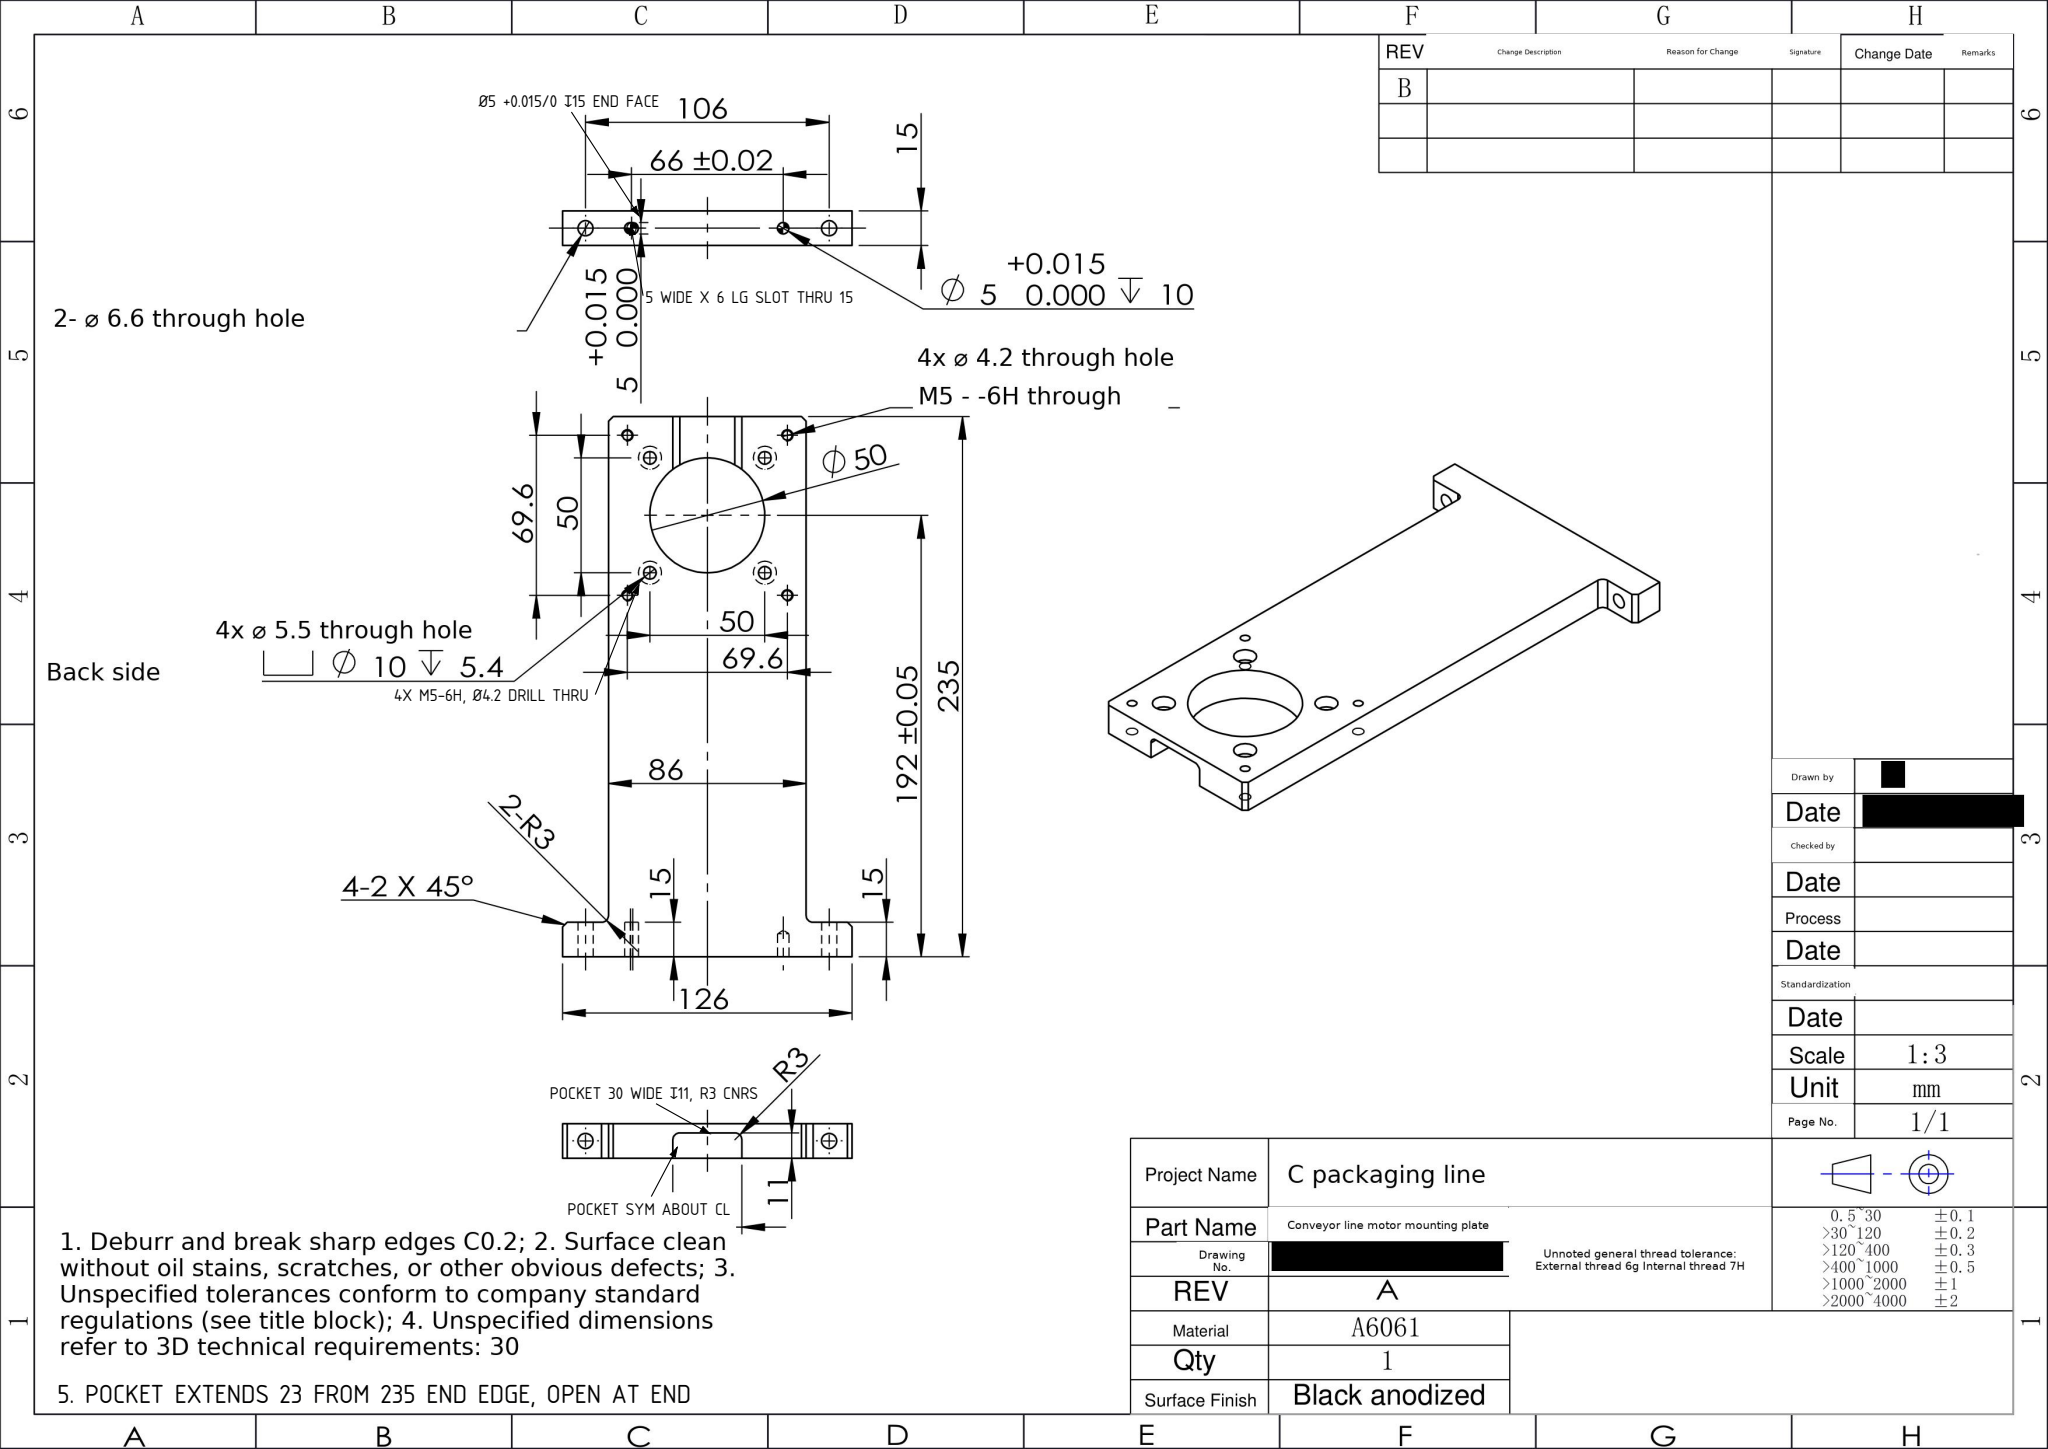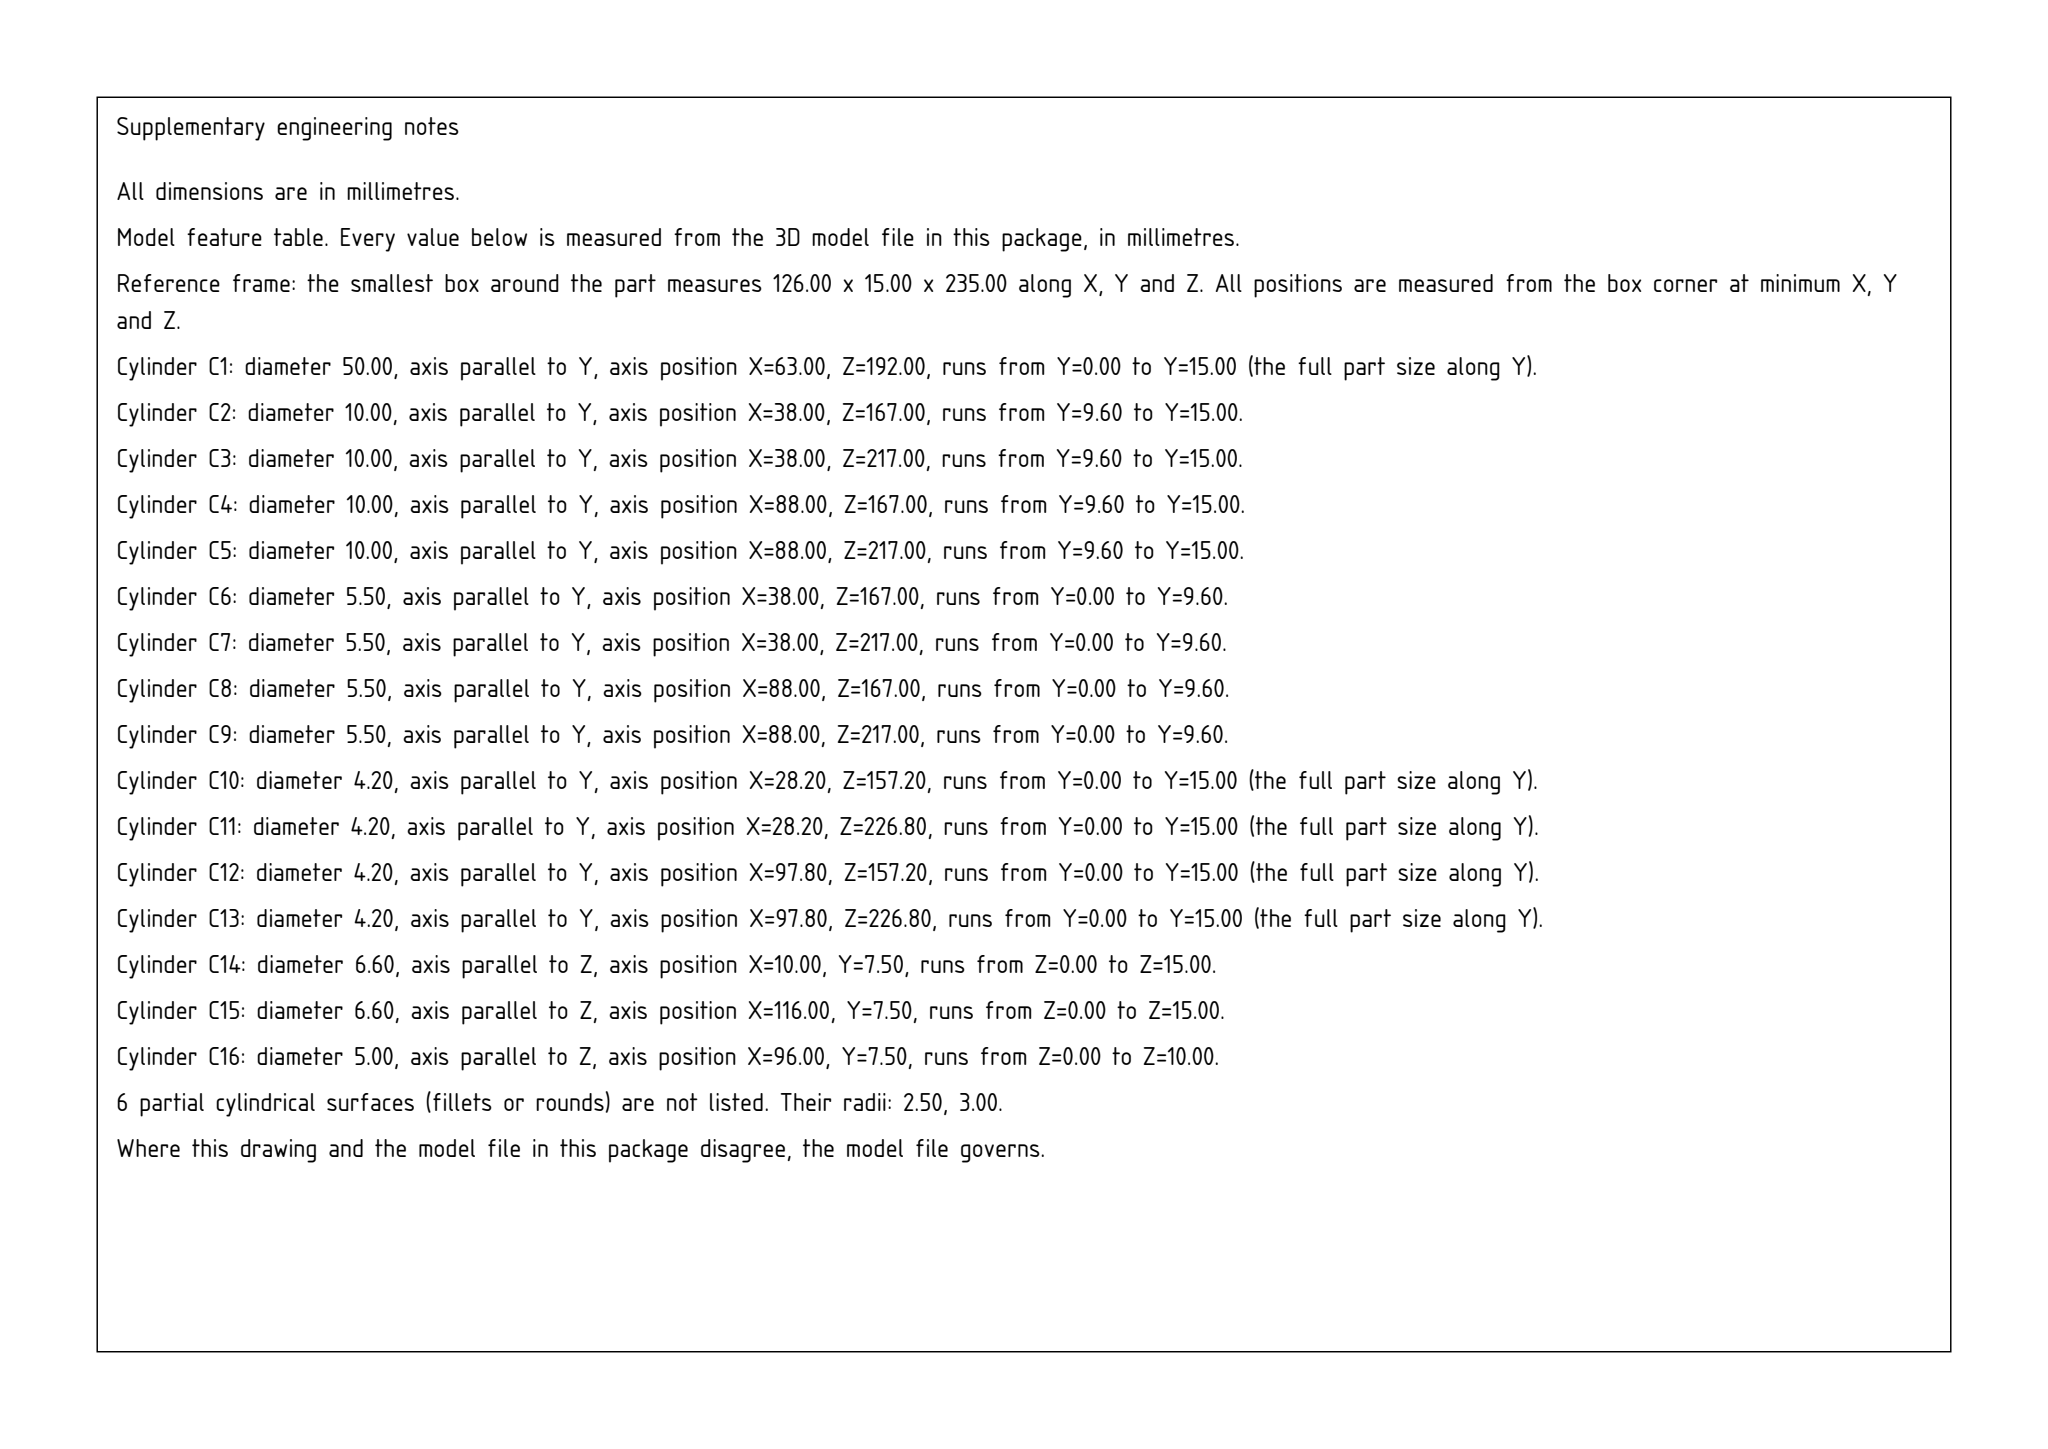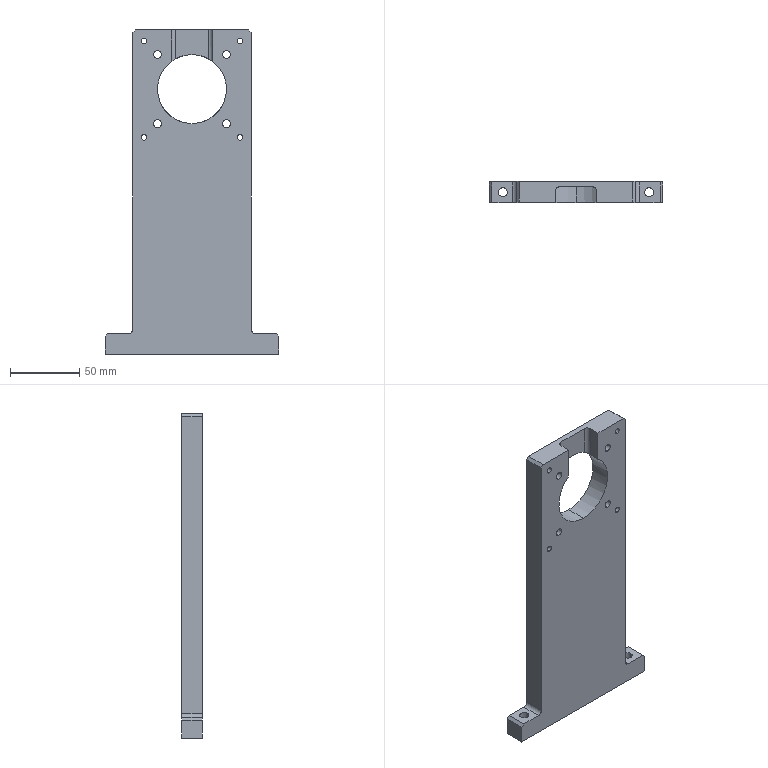Part | SolidWorks | mm | material A6061 | 1 solid | 65 faces | box 126 x 15 x 235 mm | volume 271215 mm3 | cylinder 39 | plane 24 | cone 2 | commonest cylinder face diameters 10 x8 5.5 x8 4.2 x8 5 x5 6.6 x4 6 x4 50 x2
Drawing notes:
Ø5 H7 HOLE IS SLOT: 5 WIDE x 6 LG THRU 15, ELONG ALONG 106 DIM | from the solid: Two 180° concave arcs Ø5, axis z, at x=29.5 & 30.5, y=7.5, z 0->15; planes y=5 & y=10 span x 29.5-30.5 (slot flanks): 5 wide x 6 long, centers 1 apart along X
POCKET AT 235 END, BACK SIDE: 30 WIDE x 11 DP, R3 CNRS | from the solid: Planes x=48 & x=78 (y 0-8, z 212-235) give 30 width; floor plane y=11 x[51,75]; R3 fillets dia 6 axis z at (51,8) and (75,8)
POCKET EXTENDS 23 FROM 235 END EDGE, OPEN AT END | from the solid: Pocket faces run z=212 to z=235 (bbox z max 235): 235-212=23
POCKET SYM ABOUT PART CL (126 WIDE) | from the solid: x 48 to 78 is centered on x=63 = half of bbox x 126
4X M5-6H THRU, Ø4.2 TAP DRILL THRU | from the solid: 4x Ø4.2 holes axis y, x=28.2/97.8, z=157.2/226.8, from y=0 to 15 (full 15 thk) = M5 tap drill
Ø5 +0.015/0 SLOT 6 LG DP 15 IN END FACE; OTHER Ø5 DP 10 | from the solid: Two 180° dia-5 arcs axis z at x=29.5 & 30.5, y=7.5, z 0-15 with end plane z=15 x[27,33] y[5,10] = 5 wide x 6 lg x 15 dp; separate Ø5 hole at x=96, y=7.5, z 0-10
build123d program:
from build123d import *

# Parameters (mm, degrees)
SKETCH1_W                                       = 86
SKETCH1_H                                       = 235
BOSS_EXTRUDE1_DEPTH                             = 15
SKETCH2_W                                       = 20
SKETCH2_H                                       = 15
BOSS_EXTRUDE2_DEPTH                             = 15
CHAMFER1_SIZE                                   = 2
F_6_6_6_6_DIAMETER_HOLE1_D                      = 6.6
CHAMFER2_SIZE                                   = 2
SKETCH6_W                                       = 65.064
SKETCH6_H                                       = 67.78
SKETCH6_W_2                                     = 26.869
SKETCH6_H_2                                     = 69.526
CUT_EXTRUDE2_DEPTH                              = 135.165
CHAMFER3_SIZE                                   = 2
F_5_0MM_DOWEL_PIN_HOLE1_D                       = 5
F_5_0MM_DOWEL_PIN_HOLE1_DEPTH                   = 10
F_5_0MM_DOWEL_PIN_HOLE1_TIP                     = 1.502
FILLET1_R                                       = 3
CUT_EXTRUDE3_DEPTH                              = 135.165
CUT_EXTRUDE3_DEPTH_BACK                         = 135.165
SKETCH12_R                                      = 25
M5_TAPPED_HOLE1_D                               = 4.2
M5_HEX_SOCKET_HEAD_CAP_SCREW_CBORE1_D           = 5.5
M5_HEX_SOCKET_HEAD_CAP_SCREW_CBORE1_CBORE_D     = 10
M5_HEX_SOCKET_HEAD_CAP_SCREW_CBORE1_CBORE_DEPTH = 5.4
CUT_EXTRUDE4_DEPTH                              = 32
CUT_EXTRUDE5_DEPTH                              = 25
CUT_EXTRUDE6_DEPTH                              = 15


with BuildPart() as part:
    # Sketch1 → Boss-Extrude1 (new body)
    with BuildSketch(Plane(origin=(0, 0, 0), x_dir=(1, 0, 0), z_dir=(0, 1, 0))):
        Rectangle(SKETCH1_W, SKETCH1_H)
    extrude(amount=BOSS_EXTRUDE1_DEPTH)

    # Sketch2 → Boss-Extrude2 (add)
    with BuildSketch(Plane(origin=(0, 15, 0), x_dir=(1, 0, 0), z_dir=(0, 1, 0))):
        with Locations((-53, -110)):
            Rectangle(SKETCH2_W, SKETCH2_H)
        with Locations((53, -110)):
            Rectangle(SKETCH2_W, SKETCH2_H)
    boss_extrude2 = extrude(amount=-BOSS_EXTRUDE2_DEPTH)

    # Chamfer1
    chamfer1_edges = [part.edges().sort_by_distance(p)[0] for p in [
        (-63, 7.5, 102.5),
        (63, 7.5, 102.5),
    ]]
    chamfer(chamfer1_edges, length=CHAMFER1_SIZE)

    # 6.6 _6.6_ Diameter Hole1 (through all)
    with Locations(Plane(origin=(0, 0, 102.5), x_dir=(-1, 0, 0), z_dir=(0, 0, -1))):
        with Locations((53, 7.5), (-53, 7.5)):
            f_6_6_6_6_diameter_hole1 = Hole(F_6_6_6_6_DIAMETER_HOLE1_D / 2)

    # Mirror1: Boss-Extrude2, 6.6 _6.6_ Diameter Hole1 across plane
    add(boss_extrude2.mirror(Plane.XY))
    add(f_6_6_6_6_diameter_hole1.mirror(Plane.XY), mode=Mode.SUBTRACT)

    # Chamfer2
    chamfer2_edges = [part.edges().sort_by_distance(p)[0] for p in [
        (-63, 7.5, -102.5),
        (63, 7.5, -102.5),
    ]]
    chamfer(chamfer2_edges, length=CHAMFER2_SIZE)

    # Sketch6 → Cut-Extrude2 (cut, through all)
    with BuildSketch(Plane(origin=(0, 15, 0), x_dir=(1, 0, 0), z_dir=(0, 1, 0))):
        with Locations((75.532, -83.61)):
            Rectangle(SKETCH6_W, SKETCH6_H)
        with Locations((-56.434, -82.737)):
            Rectangle(SKETCH6_W_2, SKETCH6_H_2)
    extrude(amount=-CUT_EXTRUDE2_DEPTH, mode=Mode.SUBTRACT)

    # Chamfer3
    chamfer3_edges = [part.edges().sort_by_distance(p)[0] for p in [
        (43, 7.5, 117.5),
        (-43, 7.5, 117.5),
    ]]
    chamfer(chamfer3_edges, length=CHAMFER3_SIZE)

    # 5.0mm Dowel Pin Hole1
    with Locations(Plane(origin=(0, 0, -117.5), x_dir=(-1, 0, 0), z_dir=(0, 0, -1))):
        with Locations((-33, 7.5), (33, 7.5)):
            Hole(F_5_0MM_DOWEL_PIN_HOLE1_D / 2, depth=F_5_0MM_DOWEL_PIN_HOLE1_DEPTH)
            with Locations((0, 0, -(F_5_0MM_DOWEL_PIN_HOLE1_DEPTH + F_5_0MM_DOWEL_PIN_HOLE1_TIP / 2))):  # 118° drill point
                Cone(0, F_5_0MM_DOWEL_PIN_HOLE1_D / 2, F_5_0MM_DOWEL_PIN_HOLE1_TIP, mode=Mode.SUBTRACT)

    # Fillet1
    fillet1_edges = [part.edges().sort_by_distance(p)[0] for p in [
        (-43, 7.5, -102.5),
        (43, 7.5, -102.5),
    ]]
    fillet(fillet1_edges, radius=FILLET1_R)

    # Sketch12 → Cut-Extrude3 (cut, two sides: drawn at the far end of the back side and taken through both)
    with BuildSketch(Plane.XZ.offset(-CUT_EXTRUDE3_DEPTH_BACK)):
        with Locations(Location((0, 74.5, 0), (0, 0, 270))):
            Circle(SKETCH12_R)
    extrude(amount=CUT_EXTRUDE3_DEPTH + CUT_EXTRUDE3_DEPTH_BACK, mode=Mode.SUBTRACT)

    # M5 Tapped Hole1 (through all)
    with Locations(Plane(origin=(0, 0, 0), x_dir=(-1, 0, 0), z_dir=(0, -1, 0))):
        with Locations((34.8, -109.3), (-34.8, -109.3), (34.8, -39.7), (-34.8, -39.7)):
            Hole(M5_TAPPED_HOLE1_D / 2)

    # M5 Hex Socket Head Cap Screw CBORE1 (through all)
    with Locations(Plane(origin=(0, 15, 0), x_dir=(1, 0, 0), z_dir=(0, 1, 0))):
        with Locations((25, -99.5), (-25, -99.5), (-25, -49.5), (25, -49.5)):
            CounterBoreHole(M5_HEX_SOCKET_HEAD_CAP_SCREW_CBORE1_D / 2, M5_HEX_SOCKET_HEAD_CAP_SCREW_CBORE1_CBORE_D / 2, M5_HEX_SOCKET_HEAD_CAP_SCREW_CBORE1_CBORE_DEPTH)

    # Sketch17 → Cut-Extrude4 (cut)
    with BuildSketch(Plane.XY.offset(117.5)):
        with BuildLine():
            Line((-4, -1.061), (-4, 7))
            ThreePointArc((-4, 7), (0, 11), (4, 7))
            Line((4, 7), (4, -1.061))
            ThreePointArc((4, -1.061), (0, -5.061), (-4, -1.061))
        make_face()
    extrude(amount=-CUT_EXTRUDE4_DEPTH, mode=Mode.SUBTRACT)

    # Sketch18 → Cut-Extrude5 (cut)
    with BuildSketch(Plane.XY.offset(117.5)):
        with BuildLine():
            Line((-12, 11), (12, 11))
            ThreePointArc((12, 11), (14.121, 10.121), (15, 8))
            Line((15, 8), (15, -19.287))
            Line((15, -19.287), (-15, -19.287))
            Line((-15, -19.287), (-15, 8))
            ThreePointArc((-15, 8), (-14.121, 10.121), (-12, 11))
        make_face()
    extrude(amount=-CUT_EXTRUDE5_DEPTH, mode=Mode.SUBTRACT)

    # Sketch19 → Cut-Extrude6 (cut)
    with BuildSketch(Plane(origin=(0, 0, -117.5), x_dir=(-1, 0, 0), z_dir=(0, 0, -1))):
        with BuildLine():
            Line((33.5, 5), (32.5, 5))
            ThreePointArc((32.5, 5), (30, 7.5), (32.5, 10))
            Line((32.5, 10), (33.5, 10))
            ThreePointArc((33.5, 10), (36, 7.5), (33.5, 5))
        make_face()
    extrude(amount=-CUT_EXTRUDE6_DEPTH, mode=Mode.SUBTRACT)


solid = part.part